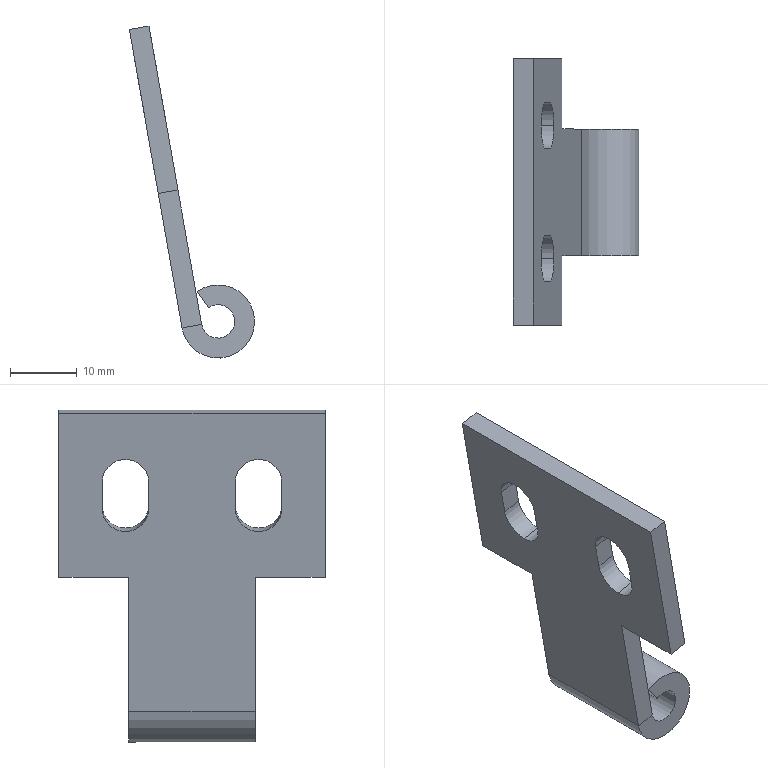Component | SolidWorks | KSHE-016.4-1_Hinge1-1 | 1 solid | 24 faces | box 18.82 x 40 x 49.87 mm | volume 4944 mm3 | plane 16 | cylinder 8 | commonest cylinder face diameters 7 x6 11 x1 5 x1
STEP:
#1=CARTESIAN_POINT('',(-12.205,5.878,2.959));
#2=VERTEX_POINT('',#1);
#3=CARTESIAN_POINT('',(-12.229,5.741,3.094));
#4=VERTEX_POINT('',#3);
#5=CARTESIAN_POINT('',(-12.229,5.878,3.094));
#6=DIRECTION('',(-0.9848,-0.,-0.1736));
#7=DIRECTION('',(0.1736,0.,-0.9848));
#8=AXIS2_PLACEMENT_3D('',#5,#6,#7);
#9=CIRCLE('',#8,0.1378);
#10=EDGE_CURVE('',#2,#4,#9,.T.);
#11=ORIENTED_EDGE('',*,*,#10,.F.);
#12=CARTESIAN_POINT('',(-12.321,5.878,2.938));
#13=VERTEX_POINT('',#12);
#14=CARTESIAN_POINT('',(-11.934,5.878,3.006));
#15=DIRECTION('',(-0.9848,-0.,-0.1736));
#16=VECTOR('',#15,39.37);
#17=LINE('',#14,#16);
#18=EDGE_CURVE('',#2,#13,#17,.T.);
#19=ORIENTED_EDGE('',*,*,#18,.T.);
#20=CARTESIAN_POINT('',(-12.345,5.741,3.074));
#21=VERTEX_POINT('',#20);
#22=CARTESIAN_POINT('',(-12.345,5.878,3.074));
#23=DIRECTION('',(-0.9848,-0.,-0.1736));
#24=DIRECTION('',(0.1736,0.,-0.9848));
#25=AXIS2_PLACEMENT_3D('',#22,#23,#24);
#26=CIRCLE('',#25,0.1378);
#27=EDGE_CURVE('',#13,#21,#26,.T.);
#28=ORIENTED_EDGE('',*,*,#27,.T.);
#29=CARTESIAN_POINT('',(-11.958,5.741,3.142));
#30=DIRECTION('',(-0.9848,-0.,-0.1736));
#31=VECTOR('',#30,39.37);
#32=LINE('',#29,#31);
#33=EDGE_CURVE('',#4,#21,#32,.T.);
#34=ORIENTED_EDGE('',*,*,#33,.F.);
#35=EDGE_LOOP('',(#11,#19,#28,#34));
#36=FACE_OUTER_BOUND('',#35,.T.);
#37=CARTESIAN_POINT('',(-11.958,5.878,3.142));
#38=DIRECTION('',(-0.9848,-0.,-0.1736));
#39=DIRECTION('',(0.1736,0.,-0.9848));
#40=AXIS2_PLACEMENT_3D('',#37,#38,#39);
#41=CYLINDRICAL_SURFACE('',#40,0.1378);
#42=ADVANCED_FACE('',(#36),#41,.F.);
#43=CARTESIAN_POINT('',(-12.205,5.091,2.959));
#44=VERTEX_POINT('',#43);
#45=CARTESIAN_POINT('',(-12.229,4.953,3.094));
#46=VERTEX_POINT('',#45);
#47=CARTESIAN_POINT('',(-12.229,5.091,3.094));
#48=DIRECTION('',(-0.9848,-0.,-0.1736));
#49=DIRECTION('',(0.1736,0.,-0.9848));
#50=AXIS2_PLACEMENT_3D('',#47,#48,#49);
#51=CIRCLE('',#50,0.1378);
#52=EDGE_CURVE('',#44,#46,#51,.T.);
#53=ORIENTED_EDGE('',*,*,#52,.F.);
#54=CARTESIAN_POINT('',(-12.321,5.091,2.938));
#55=VERTEX_POINT('',#54);
#56=CARTESIAN_POINT('',(-11.934,5.091,3.006));
#57=DIRECTION('',(-0.9848,-0.,-0.1736));
#58=VECTOR('',#57,39.37);
#59=LINE('',#56,#58);
#60=EDGE_CURVE('',#44,#55,#59,.T.);
#61=ORIENTED_EDGE('',*,*,#60,.T.);
#62=CARTESIAN_POINT('',(-12.345,4.953,3.074));
#63=VERTEX_POINT('',#62);
#64=CARTESIAN_POINT('',(-12.345,5.091,3.074));
#65=DIRECTION('',(-0.9848,-0.,-0.1736));
#66=DIRECTION('',(0.1736,0.,-0.9848));
#67=AXIS2_PLACEMENT_3D('',#64,#65,#66);
#68=CIRCLE('',#67,0.1378);
#69=EDGE_CURVE('',#55,#63,#68,.T.);
#70=ORIENTED_EDGE('',*,*,#69,.T.);
#71=CARTESIAN_POINT('',(-11.958,4.953,3.142));
#72=DIRECTION('',(-0.9848,-0.,-0.1736));
#73=VECTOR('',#72,39.37);
#74=LINE('',#71,#73);
#75=EDGE_CURVE('',#46,#63,#74,.T.);
#76=ORIENTED_EDGE('',*,*,#75,.F.);
#77=EDGE_LOOP('',(#53,#61,#70,#76));
#78=FACE_OUTER_BOUND('',#77,.T.);
#79=CARTESIAN_POINT('',(-11.958,5.091,3.142));
#80=DIRECTION('',(-0.9848,-0.,-0.1736));
#81=DIRECTION('',(0.1736,0.,-0.9848));
#82=AXIS2_PLACEMENT_3D('',#79,#80,#81);
#83=CYLINDRICAL_SURFACE('',#82,0.1378);
#84=ADVANCED_FACE('',(#78),#83,.F.);
#85=CARTESIAN_POINT('',(-12.274,6.272,2.667));
#86=VERTEX_POINT('',#85);
#87=CARTESIAN_POINT('',(-12.157,6.272,2.687));
#88=VERTEX_POINT('',#87);
#89=CARTESIAN_POINT('',(-12.157,6.272,2.687));
#90=DIRECTION('',(0.9848,0.,0.1736));
#91=VECTOR('',#90,39.37);
#92=LINE('',#89,#91);
#93=EDGE_CURVE('',#86,#88,#92,.T.);
#94=ORIENTED_EDGE('',*,*,#93,.F.);
#95=CARTESIAN_POINT('',(-12.445,6.272,3.636));
#96=VERTEX_POINT('',#95);
#97=CARTESIAN_POINT('',(-12.445,6.272,3.636));
#98=DIRECTION('',(0.1736,-0.,-0.9848));
#99=VECTOR('',#98,39.37);
#100=LINE('',#97,#99);
#101=EDGE_CURVE('',#96,#86,#100,.T.);
#102=ORIENTED_EDGE('',*,*,#101,.F.);
#103=CARTESIAN_POINT('',(-12.328,6.272,3.656));
#104=VERTEX_POINT('',#103);
#105=CARTESIAN_POINT('',(-12.328,6.272,3.656));
#106=DIRECTION('',(-0.9848,-0.,-0.1736));
#107=VECTOR('',#106,39.37);
#108=LINE('',#105,#107);
#109=EDGE_CURVE('',#104,#96,#108,.T.);
#110=ORIENTED_EDGE('',*,*,#109,.F.);
#111=CARTESIAN_POINT('',(-12.328,6.272,3.656));
#112=DIRECTION('',(0.1736,-0.,-0.9848));
#113=VECTOR('',#112,39.37);
#114=LINE('',#111,#113);
#115=EDGE_CURVE('',#104,#88,#114,.T.);
#116=ORIENTED_EDGE('',*,*,#115,.T.);
#117=EDGE_LOOP('',(#94,#102,#110,#116));
#118=FACE_OUTER_BOUND('',#117,.T.);
#119=CARTESIAN_POINT('',(-12.328,6.272,3.656));
#120=DIRECTION('',(-0.,1.,-0.));
#121=DIRECTION('',(0.9848,0.,0.1736));
#122=AXIS2_PLACEMENT_3D('',#119,#120,#121);
#123=PLANE('',#122);
#124=ADVANCED_FACE('',(#118),#123,.T.);
#125=CARTESIAN_POINT('',(-12.445,4.697,3.636));
#126=VERTEX_POINT('',#125);
#127=CARTESIAN_POINT('',(-12.445,4.697,3.636));
#128=DIRECTION('',(-0.,1.,-0.));
#129=VECTOR('',#128,39.37);
#130=LINE('',#127,#129);
#131=EDGE_CURVE('',#126,#96,#130,.T.);
#132=ORIENTED_EDGE('',*,*,#131,.F.);
#133=CARTESIAN_POINT('',(-12.328,4.697,3.656));
#134=VERTEX_POINT('',#133);
#135=CARTESIAN_POINT('',(-12.328,4.697,3.656));
#136=DIRECTION('',(-0.9848,-0.,-0.1736));
#137=VECTOR('',#136,39.37);
#138=LINE('',#135,#137);
#139=EDGE_CURVE('',#134,#126,#138,.T.);
#140=ORIENTED_EDGE('',*,*,#139,.F.);
#141=CARTESIAN_POINT('',(-12.328,4.697,3.656));
#142=DIRECTION('',(-0.,1.,-0.));
#143=VECTOR('',#142,39.37);
#144=LINE('',#141,#143);
#145=EDGE_CURVE('',#134,#104,#144,.T.);
#146=ORIENTED_EDGE('',*,*,#145,.T.);
#147=ORIENTED_EDGE('',*,*,#109,.T.);
#148=EDGE_LOOP('',(#132,#140,#146,#147));
#149=FACE_OUTER_BOUND('',#148,.T.);
#150=CARTESIAN_POINT('',(-12.328,4.697,3.656));
#151=DIRECTION('',(-0.1736,0.,0.9848));
#152=DIRECTION('',(-0.,1.,-0.));
#153=AXIS2_PLACEMENT_3D('',#150,#151,#152);
#154=PLANE('',#153);
#155=ADVANCED_FACE('',(#149),#154,.T.);
#156=CARTESIAN_POINT('',(-12.157,4.697,2.687));
#157=VERTEX_POINT('',#156);
#158=CARTESIAN_POINT('',(-12.274,4.697,2.667));
#159=VERTEX_POINT('',#158);
#160=CARTESIAN_POINT('',(-12.157,4.697,2.687));
#161=DIRECTION('',(-0.9848,-0.,-0.1736));
#162=VECTOR('',#161,39.37);
#163=LINE('',#160,#162);
#164=EDGE_CURVE('',#157,#159,#163,.T.);
#165=ORIENTED_EDGE('',*,*,#164,.F.);
#166=CARTESIAN_POINT('',(-12.328,4.697,3.656));
#167=DIRECTION('',(-0.1736,0.,0.9848));
#168=VECTOR('',#167,39.37);
#169=LINE('',#166,#168);
#170=EDGE_CURVE('',#157,#134,#169,.T.);
#171=ORIENTED_EDGE('',*,*,#170,.T.);
#172=ORIENTED_EDGE('',*,*,#139,.T.);
#173=CARTESIAN_POINT('',(-12.445,4.697,3.636));
#174=DIRECTION('',(-0.1736,0.,0.9848));
#175=VECTOR('',#174,39.37);
#176=LINE('',#173,#175);
#177=EDGE_CURVE('',#159,#126,#176,.T.);
#178=ORIENTED_EDGE('',*,*,#177,.F.);
#179=EDGE_LOOP('',(#165,#171,#172,#178));
#180=FACE_OUTER_BOUND('',#179,.T.);
#181=CARTESIAN_POINT('',(-12.328,4.697,3.656));
#182=DIRECTION('',(0.,-1.,0.));
#183=DIRECTION('',(-0.9848,-0.,-0.1736));
#184=AXIS2_PLACEMENT_3D('',#181,#182,#183);
#185=PLANE('',#184);
#186=ADVANCED_FACE('',(#180),#185,.T.);
#187=CARTESIAN_POINT('',(-12.256,5.741,3.249));
#188=VERTEX_POINT('',#187);
#189=CARTESIAN_POINT('',(-12.154,5.741,2.668));
#190=DIRECTION('',(-0.1736,0.,0.9848));
#191=VECTOR('',#190,39.37);
#192=LINE('',#189,#191);
#193=EDGE_CURVE('',#4,#188,#192,.T.);
#194=ORIENTED_EDGE('',*,*,#193,.T.);
#195=CARTESIAN_POINT('',(-12.256,6.016,3.249));
#196=VERTEX_POINT('',#195);
#197=CARTESIAN_POINT('',(-12.256,5.878,3.249));
#198=DIRECTION('',(-0.9848,-0.,-0.1736));
#199=DIRECTION('',(0.1736,0.,-0.9848));
#200=AXIS2_PLACEMENT_3D('',#197,#198,#199);
#201=CIRCLE('',#200,0.1378);
#202=EDGE_CURVE('',#188,#196,#201,.T.);
#203=ORIENTED_EDGE('',*,*,#202,.T.);
#204=CARTESIAN_POINT('',(-12.229,6.016,3.094));
#205=VERTEX_POINT('',#204);
#206=CARTESIAN_POINT('',(-12.154,6.016,2.668));
#207=DIRECTION('',(0.1736,-0.,-0.9848));
#208=VECTOR('',#207,39.37);
#209=LINE('',#206,#208);
#210=EDGE_CURVE('',#196,#205,#209,.T.);
#211=ORIENTED_EDGE('',*,*,#210,.T.);
#212=CARTESIAN_POINT('',(-12.229,5.878,3.094));
#213=DIRECTION('',(-0.9848,-0.,-0.1736));
#214=DIRECTION('',(0.1736,0.,-0.9848));
#215=AXIS2_PLACEMENT_3D('',#212,#213,#214);
#216=CIRCLE('',#215,0.1378);
#217=EDGE_CURVE('',#205,#2,#216,.T.);
#218=ORIENTED_EDGE('',*,*,#217,.T.);
#219=ORIENTED_EDGE('',*,*,#10,.T.);
#220=EDGE_LOOP('',(#194,#203,#211,#218,#219));
#221=FACE_BOUND('',#220,.T.);
#222=CARTESIAN_POINT('',(-12.256,4.953,3.249));
#223=VERTEX_POINT('',#222);
#224=CARTESIAN_POINT('',(-12.154,4.953,2.668));
#225=DIRECTION('',(-0.1736,0.,0.9848));
#226=VECTOR('',#225,39.37);
#227=LINE('',#224,#226);
#228=EDGE_CURVE('',#46,#223,#227,.T.);
#229=ORIENTED_EDGE('',*,*,#228,.T.);
#230=CARTESIAN_POINT('',(-12.256,5.229,3.249));
#231=VERTEX_POINT('',#230);
#232=CARTESIAN_POINT('',(-12.256,5.091,3.249));
#233=DIRECTION('',(-0.9848,-0.,-0.1736));
#234=DIRECTION('',(0.1736,0.,-0.9848));
#235=AXIS2_PLACEMENT_3D('',#232,#233,#234);
#236=CIRCLE('',#235,0.1378);
#237=EDGE_CURVE('',#223,#231,#236,.T.);
#238=ORIENTED_EDGE('',*,*,#237,.T.);
#239=CARTESIAN_POINT('',(-12.229,5.229,3.094));
#240=VERTEX_POINT('',#239);
#241=CARTESIAN_POINT('',(-12.154,5.229,2.668));
#242=DIRECTION('',(0.1736,-0.,-0.9848));
#243=VECTOR('',#242,39.37);
#244=LINE('',#241,#243);
#245=EDGE_CURVE('',#231,#240,#244,.T.);
#246=ORIENTED_EDGE('',*,*,#245,.T.);
#247=CARTESIAN_POINT('',(-12.229,5.091,3.094));
#248=DIRECTION('',(-0.9848,-0.,-0.1736));
#249=DIRECTION('',(0.1736,0.,-0.9848));
#250=AXIS2_PLACEMENT_3D('',#247,#248,#249);
#251=CIRCLE('',#250,0.1378);
#252=EDGE_CURVE('',#240,#44,#251,.T.);
#253=ORIENTED_EDGE('',*,*,#252,.T.);
#254=ORIENTED_EDGE('',*,*,#52,.T.);
#255=EDGE_LOOP('',(#229,#238,#246,#253,#254));
#256=FACE_BOUND('',#255,.T.);
#257=CARTESIAN_POINT('',(-12.157,5.111,2.687));
#258=VERTEX_POINT('',#257);
#259=CARTESIAN_POINT('',(-12.017,5.111,1.892));
#260=VERTEX_POINT('',#259);
#261=CARTESIAN_POINT('',(-12.154,5.111,2.668));
#262=DIRECTION('',(0.1736,-0.,-0.9848));
#263=VECTOR('',#262,39.37);
#264=LINE('',#261,#263);
#265=EDGE_CURVE('',#258,#260,#264,.T.);
#266=ORIENTED_EDGE('',*,*,#265,.T.);
#267=CARTESIAN_POINT('',(-12.017,5.859,1.892));
#268=VERTEX_POINT('',#267);
#269=CARTESIAN_POINT('',(-12.017,5.859,1.892));
#270=DIRECTION('',(0.,-1.,0.));
#271=VECTOR('',#270,39.37);
#272=LINE('',#269,#271);
#273=EDGE_CURVE('',#268,#260,#272,.T.);
#274=ORIENTED_EDGE('',*,*,#273,.F.);
#275=CARTESIAN_POINT('',(-12.157,5.859,2.687));
#276=VERTEX_POINT('',#275);
#277=CARTESIAN_POINT('',(-12.154,5.859,2.668));
#278=DIRECTION('',(-0.1736,0.,0.9848));
#279=VECTOR('',#278,39.37);
#280=LINE('',#277,#279);
#281=EDGE_CURVE('',#268,#276,#280,.T.);
#282=ORIENTED_EDGE('',*,*,#281,.T.);
#283=CARTESIAN_POINT('',(-12.157,5.485,2.687));
#284=DIRECTION('',(-0.,1.,-0.));
#285=VECTOR('',#284,39.37);
#286=LINE('',#283,#285);
#287=EDGE_CURVE('',#276,#88,#286,.T.);
#288=ORIENTED_EDGE('',*,*,#287,.T.);
#289=ORIENTED_EDGE('',*,*,#115,.F.);
#290=ORIENTED_EDGE('',*,*,#145,.F.);
#291=ORIENTED_EDGE('',*,*,#170,.F.);
#292=CARTESIAN_POINT('',(-12.157,5.485,2.687));
#293=DIRECTION('',(-0.,1.,-0.));
#294=VECTOR('',#293,39.37);
#295=LINE('',#292,#294);
#296=EDGE_CURVE('',#157,#258,#295,.T.);
#297=ORIENTED_EDGE('',*,*,#296,.T.);
#298=EDGE_LOOP('',(#266,#274,#282,#288,#289,#290,#291,#297));
#299=FACE_OUTER_BOUND('',#298,.T.);
#300=CARTESIAN_POINT('',(-12.154,5.485,2.668));
#301=DIRECTION('',(-0.9848,-0.,-0.1736));
#302=DIRECTION('',(0.1736,-0.,-0.9848));
#303=AXIS2_PLACEMENT_3D('',#300,#301,#302);
#304=PLANE('',#303);
#305=ADVANCED_FACE('',(#221,#256,#299),#304,.F.);
#306=CARTESIAN_POINT('',(-12.373,5.741,3.229));
#307=VERTEX_POINT('',#306);
#308=CARTESIAN_POINT('',(-12.373,6.016,3.229));
#309=VERTEX_POINT('',#308);
#310=CARTESIAN_POINT('',(-12.373,5.878,3.229));
#311=DIRECTION('',(-0.9848,-0.,-0.1736));
#312=DIRECTION('',(0.1736,0.,-0.9848));
#313=AXIS2_PLACEMENT_3D('',#310,#311,#312);
#314=CIRCLE('',#313,0.1378);
#315=EDGE_CURVE('',#307,#309,#314,.T.);
#316=ORIENTED_EDGE('',*,*,#315,.F.);
#317=CARTESIAN_POINT('',(-12.373,5.741,3.229));
#318=DIRECTION('',(-0.1736,0.,0.9848));
#319=VECTOR('',#318,39.37);
#320=LINE('',#317,#319);
#321=EDGE_CURVE('',#21,#307,#320,.T.);
#322=ORIENTED_EDGE('',*,*,#321,.F.);
#323=ORIENTED_EDGE('',*,*,#27,.F.);
#324=CARTESIAN_POINT('',(-12.345,6.016,3.074));
#325=VERTEX_POINT('',#324);
#326=CARTESIAN_POINT('',(-12.345,5.878,3.074));
#327=DIRECTION('',(-0.9848,-0.,-0.1736));
#328=DIRECTION('',(0.1736,0.,-0.9848));
#329=AXIS2_PLACEMENT_3D('',#326,#327,#328);
#330=CIRCLE('',#329,0.1378);
#331=EDGE_CURVE('',#325,#13,#330,.T.);
#332=ORIENTED_EDGE('',*,*,#331,.F.);
#333=CARTESIAN_POINT('',(-12.373,6.016,3.229));
#334=DIRECTION('',(0.1736,-0.,-0.9848));
#335=VECTOR('',#334,39.37);
#336=LINE('',#333,#335);
#337=EDGE_CURVE('',#309,#325,#336,.T.);
#338=ORIENTED_EDGE('',*,*,#337,.F.);
#339=EDGE_LOOP('',(#316,#322,#323,#332,#338));
#340=FACE_BOUND('',#339,.T.);
#341=CARTESIAN_POINT('',(-12.373,4.953,3.229));
#342=VERTEX_POINT('',#341);
#343=CARTESIAN_POINT('',(-12.373,5.229,3.229));
#344=VERTEX_POINT('',#343);
#345=CARTESIAN_POINT('',(-12.373,5.091,3.229));
#346=DIRECTION('',(-0.9848,-0.,-0.1736));
#347=DIRECTION('',(0.1736,0.,-0.9848));
#348=AXIS2_PLACEMENT_3D('',#345,#346,#347);
#349=CIRCLE('',#348,0.1378);
#350=EDGE_CURVE('',#342,#344,#349,.T.);
#351=ORIENTED_EDGE('',*,*,#350,.F.);
#352=CARTESIAN_POINT('',(-12.373,4.953,3.229));
#353=DIRECTION('',(-0.1736,0.,0.9848));
#354=VECTOR('',#353,39.37);
#355=LINE('',#352,#354);
#356=EDGE_CURVE('',#63,#342,#355,.T.);
#357=ORIENTED_EDGE('',*,*,#356,.F.);
#358=ORIENTED_EDGE('',*,*,#69,.F.);
#359=CARTESIAN_POINT('',(-12.345,5.229,3.074));
#360=VERTEX_POINT('',#359);
#361=CARTESIAN_POINT('',(-12.345,5.091,3.074));
#362=DIRECTION('',(-0.9848,-0.,-0.1736));
#363=DIRECTION('',(0.1736,0.,-0.9848));
#364=AXIS2_PLACEMENT_3D('',#361,#362,#363);
#365=CIRCLE('',#364,0.1378);
#366=EDGE_CURVE('',#360,#55,#365,.T.);
#367=ORIENTED_EDGE('',*,*,#366,.F.);
#368=CARTESIAN_POINT('',(-12.373,5.229,3.229));
#369=DIRECTION('',(0.1736,-0.,-0.9848));
#370=VECTOR('',#369,39.37);
#371=LINE('',#368,#370);
#372=EDGE_CURVE('',#344,#360,#371,.T.);
#373=ORIENTED_EDGE('',*,*,#372,.F.);
#374=EDGE_LOOP('',(#351,#357,#358,#367,#373));
#375=FACE_BOUND('',#374,.T.);
#376=CARTESIAN_POINT('',(-12.133,5.859,1.872));
#377=VERTEX_POINT('',#376);
#378=CARTESIAN_POINT('',(-12.133,5.111,1.872));
#379=VERTEX_POINT('',#378);
#380=CARTESIAN_POINT('',(-12.133,5.859,1.872));
#381=DIRECTION('',(0.,-1.,0.));
#382=VECTOR('',#381,39.37);
#383=LINE('',#380,#382);
#384=EDGE_CURVE('',#377,#379,#383,.T.);
#385=ORIENTED_EDGE('',*,*,#384,.T.);
#386=CARTESIAN_POINT('',(-12.274,5.111,2.667));
#387=VERTEX_POINT('',#386);
#388=CARTESIAN_POINT('',(-12.274,5.111,2.667));
#389=DIRECTION('',(0.1736,-0.,-0.9848));
#390=VECTOR('',#389,39.37);
#391=LINE('',#388,#390);
#392=EDGE_CURVE('',#387,#379,#391,.T.);
#393=ORIENTED_EDGE('',*,*,#392,.F.);
#394=CARTESIAN_POINT('',(-12.274,5.485,2.667));
#395=DIRECTION('',(-0.,1.,-0.));
#396=VECTOR('',#395,39.37);
#397=LINE('',#394,#396);
#398=EDGE_CURVE('',#159,#387,#397,.T.);
#399=ORIENTED_EDGE('',*,*,#398,.F.);
#400=ORIENTED_EDGE('',*,*,#177,.T.);
#401=ORIENTED_EDGE('',*,*,#131,.T.);
#402=ORIENTED_EDGE('',*,*,#101,.T.);
#403=CARTESIAN_POINT('',(-12.274,5.859,2.667));
#404=VERTEX_POINT('',#403);
#405=CARTESIAN_POINT('',(-12.274,5.859,2.667));
#406=DIRECTION('',(-0.,1.,-0.));
#407=VECTOR('',#406,39.37);
#408=LINE('',#405,#407);
#409=EDGE_CURVE('',#404,#86,#408,.T.);
#410=ORIENTED_EDGE('',*,*,#409,.F.);
#411=CARTESIAN_POINT('',(-12.27,5.859,2.647));
#412=DIRECTION('',(-0.1736,0.,0.9848));
#413=VECTOR('',#412,39.37);
#414=LINE('',#411,#413);
#415=EDGE_CURVE('',#377,#404,#414,.T.);
#416=ORIENTED_EDGE('',*,*,#415,.F.);
#417=EDGE_LOOP('',(#385,#393,#399,#400,#401,#402,#410,#416));
#418=FACE_OUTER_BOUND('',#417,.T.);
#419=CARTESIAN_POINT('',(-12.27,5.485,2.647));
#420=DIRECTION('',(-0.9848,-0.,-0.1736));
#421=DIRECTION('',(0.1736,-0.,-0.9848));
#422=AXIS2_PLACEMENT_3D('',#419,#420,#421);
#423=PLANE('',#422);
#424=ADVANCED_FACE('',(#340,#375,#418),#423,.T.);
#425=ORIENTED_EDGE('',*,*,#392,.T.);
#426=CARTESIAN_POINT('',(-12.017,5.111,1.892));
#427=DIRECTION('',(-0.9848,-0.,-0.1736));
#428=VECTOR('',#427,39.37);
#429=LINE('',#426,#428);
#430=EDGE_CURVE('',#260,#379,#429,.T.);
#431=ORIENTED_EDGE('',*,*,#430,.F.);
#432=ORIENTED_EDGE('',*,*,#265,.F.);
#433=CARTESIAN_POINT('',(-11.886,5.111,2.735));
#434=DIRECTION('',(-0.9848,-0.,-0.1736));
#435=VECTOR('',#434,39.37);
#436=LINE('',#433,#435);
#437=EDGE_CURVE('',#258,#387,#436,.T.);
#438=ORIENTED_EDGE('',*,*,#437,.T.);
#439=EDGE_LOOP('',(#425,#431,#432,#438));
#440=FACE_OUTER_BOUND('',#439,.T.);
#441=CARTESIAN_POINT('',(-11.886,5.111,2.735));
#442=DIRECTION('',(-0.,1.,-0.));
#443=DIRECTION('',(0.9848,0.,0.1736));
#444=AXIS2_PLACEMENT_3D('',#441,#442,#443);
#445=PLANE('',#444);
#446=ADVANCED_FACE('',(#440),#445,.F.);
#447=ORIENTED_EDGE('',*,*,#164,.T.);
#448=ORIENTED_EDGE('',*,*,#398,.T.);
#449=ORIENTED_EDGE('',*,*,#437,.F.);
#450=ORIENTED_EDGE('',*,*,#296,.F.);
#451=EDGE_LOOP('',(#447,#448,#449,#450));
#452=FACE_OUTER_BOUND('',#451,.T.);
#453=CARTESIAN_POINT('',(-11.886,4.284,2.735));
#454=DIRECTION('',(-0.1736,0.,0.9848));
#455=DIRECTION('',(-0.9848,-0.,-0.1736));
#456=AXIS2_PLACEMENT_3D('',#453,#454,#455);
#457=PLANE('',#456);
#458=ADVANCED_FACE('',(#452),#457,.F.);
#459=ORIENTED_EDGE('',*,*,#93,.T.);
#460=ORIENTED_EDGE('',*,*,#287,.F.);
#461=CARTESIAN_POINT('',(-11.886,5.859,2.735));
#462=DIRECTION('',(-0.9848,-0.,-0.1736));
#463=VECTOR('',#462,39.37);
#464=LINE('',#461,#463);
#465=EDGE_CURVE('',#276,#404,#464,.T.);
#466=ORIENTED_EDGE('',*,*,#465,.T.);
#467=ORIENTED_EDGE('',*,*,#409,.T.);
#468=EDGE_LOOP('',(#459,#460,#466,#467));
#469=FACE_OUTER_BOUND('',#468,.T.);
#470=CARTESIAN_POINT('',(-11.886,5.859,2.735));
#471=DIRECTION('',(-0.1736,0.,0.9848));
#472=DIRECTION('',(-0.9848,-0.,-0.1736));
#473=AXIS2_PLACEMENT_3D('',#470,#471,#472);
#474=PLANE('',#473);
#475=ADVANCED_FACE('',(#469),#474,.F.);
#476=ORIENTED_EDGE('',*,*,#281,.F.);
#477=CARTESIAN_POINT('',(-12.017,5.859,1.892));
#478=DIRECTION('',(-0.9848,-0.,-0.1736));
#479=VECTOR('',#478,39.37);
#480=LINE('',#477,#479);
#481=EDGE_CURVE('',#268,#377,#480,.T.);
#482=ORIENTED_EDGE('',*,*,#481,.T.);
#483=ORIENTED_EDGE('',*,*,#415,.T.);
#484=ORIENTED_EDGE('',*,*,#465,.F.);
#485=EDGE_LOOP('',(#476,#482,#483,#484));
#486=FACE_OUTER_BOUND('',#485,.T.);
#487=CARTESIAN_POINT('',(-11.886,5.859,2.735));
#488=DIRECTION('',(0.,-1.,0.));
#489=DIRECTION('',(-0.9848,-0.,-0.1736));
#490=AXIS2_PLACEMENT_3D('',#487,#488,#489);
#491=PLANE('',#490);
#492=ADVANCED_FACE('',(#486),#491,.F.);
#493=CARTESIAN_POINT('',(-11.977,5.859,1.99));
#494=VERTEX_POINT('',#493);
#495=CARTESIAN_POINT('',(-12.044,5.859,2.087));
#496=VERTEX_POINT('',#495);
#497=CARTESIAN_POINT('',(-11.977,5.859,1.99));
#498=DIRECTION('',(-0.5736,-0.,0.8192));
#499=VECTOR('',#498,39.37);
#500=LINE('',#497,#499);
#501=EDGE_CURVE('',#494,#496,#500,.T.);
#502=ORIENTED_EDGE('',*,*,#501,.F.);
#503=CARTESIAN_POINT('',(-11.977,5.111,1.99));
#504=VERTEX_POINT('',#503);
#505=CARTESIAN_POINT('',(-11.977,5.859,1.99));
#506=DIRECTION('',(-0.,1.,-0.));
#507=VECTOR('',#506,39.37);
#508=LINE('',#505,#507);
#509=EDGE_CURVE('',#504,#494,#508,.T.);
#510=ORIENTED_EDGE('',*,*,#509,.F.);
#511=CARTESIAN_POINT('',(-12.044,5.111,2.087));
#512=VERTEX_POINT('',#511);
#513=CARTESIAN_POINT('',(-11.977,5.111,1.99));
#514=DIRECTION('',(-0.5736,-0.,0.8192));
#515=VECTOR('',#514,39.37);
#516=LINE('',#513,#515);
#517=EDGE_CURVE('',#504,#512,#516,.T.);
#518=ORIENTED_EDGE('',*,*,#517,.T.);
#519=CARTESIAN_POINT('',(-12.044,5.859,2.087));
#520=DIRECTION('',(-0.,1.,-0.));
#521=VECTOR('',#520,39.37);
#522=LINE('',#519,#521);
#523=EDGE_CURVE('',#512,#496,#522,.T.);
#524=ORIENTED_EDGE('',*,*,#523,.T.);
#525=EDGE_LOOP('',(#502,#510,#518,#524));
#526=FACE_OUTER_BOUND('',#525,.T.);
#527=CARTESIAN_POINT('',(-11.977,5.485,1.99));
#528=DIRECTION('',(0.8192,0.,0.5736));
#529=DIRECTION('',(-0.,1.,-0.));
#530=AXIS2_PLACEMENT_3D('',#527,#528,#529);
#531=PLANE('',#530);
#532=ADVANCED_FACE('',(#526),#531,.F.);
#533=ORIENTED_EDGE('',*,*,#517,.F.);
#534=CARTESIAN_POINT('',(-11.92,5.111,1.909));
#535=DIRECTION('',(0.,-1.,0.));
#536=DIRECTION('',(0.9848,0.,0.1736));
#537=AXIS2_PLACEMENT_3D('',#534,#535,#536);
#538=CIRCLE('',#537,0.09843);
#539=EDGE_CURVE('',#260,#504,#538,.T.);
#540=ORIENTED_EDGE('',*,*,#539,.F.);
#541=ORIENTED_EDGE('',*,*,#430,.T.);
#542=CARTESIAN_POINT('',(-11.92,5.111,1.909));
#543=DIRECTION('',(0.,-1.,0.));
#544=DIRECTION('',(0.9848,0.,0.1736));
#545=AXIS2_PLACEMENT_3D('',#542,#543,#544);
#546=CIRCLE('',#545,0.2165);
#547=EDGE_CURVE('',#379,#512,#546,.T.);
#548=ORIENTED_EDGE('',*,*,#547,.T.);
#549=EDGE_LOOP('',(#533,#540,#541,#548));
#550=FACE_OUTER_BOUND('',#549,.T.);
#551=CARTESIAN_POINT('',(-11.92,5.111,1.909));
#552=DIRECTION('',(0.,-1.,0.));
#553=DIRECTION('',(-0.9848,-0.,-0.1736));
#554=AXIS2_PLACEMENT_3D('',#551,#552,#553);
#555=PLANE('',#554);
#556=ADVANCED_FACE('',(#550),#555,.T.);
#557=CARTESIAN_POINT('',(-11.92,5.859,1.909));
#558=DIRECTION('',(-0.,1.,-0.));
#559=DIRECTION('',(0.9848,0.,0.1736));
#560=AXIS2_PLACEMENT_3D('',#557,#558,#559);
#561=CIRCLE('',#560,0.09843);
#562=EDGE_CURVE('',#494,#268,#561,.T.);
#563=ORIENTED_EDGE('',*,*,#562,.F.);
#564=ORIENTED_EDGE('',*,*,#501,.T.);
#565=CARTESIAN_POINT('',(-11.92,5.859,1.909));
#566=DIRECTION('',(-0.,1.,-0.));
#567=DIRECTION('',(0.9848,0.,0.1736));
#568=AXIS2_PLACEMENT_3D('',#565,#566,#567);
#569=CIRCLE('',#568,0.2165);
#570=EDGE_CURVE('',#496,#377,#569,.T.);
#571=ORIENTED_EDGE('',*,*,#570,.T.);
#572=ORIENTED_EDGE('',*,*,#481,.F.);
#573=EDGE_LOOP('',(#563,#564,#571,#572));
#574=FACE_OUTER_BOUND('',#573,.T.);
#575=CARTESIAN_POINT('',(-11.92,5.859,1.909));
#576=DIRECTION('',(0.,-1.,0.));
#577=DIRECTION('',(-0.9848,-0.,-0.1736));
#578=AXIS2_PLACEMENT_3D('',#575,#576,#577);
#579=PLANE('',#578);
#580=ADVANCED_FACE('',(#574),#579,.F.);
#581=ORIENTED_EDGE('',*,*,#384,.F.);
#582=ORIENTED_EDGE('',*,*,#570,.F.);
#583=ORIENTED_EDGE('',*,*,#523,.F.);
#584=ORIENTED_EDGE('',*,*,#547,.F.);
#585=EDGE_LOOP('',(#581,#582,#583,#584));
#586=FACE_OUTER_BOUND('',#585,.T.);
#587=CARTESIAN_POINT('',(-11.92,5.859,1.909));
#588=DIRECTION('',(-0.,1.,-0.));
#589=DIRECTION('',(-0.5736,0.,0.8192));
#590=AXIS2_PLACEMENT_3D('',#587,#588,#589);
#591=CYLINDRICAL_SURFACE('',#590,0.2165);
#592=ADVANCED_FACE('',(#586),#591,.T.);
#593=ORIENTED_EDGE('',*,*,#273,.T.);
#594=ORIENTED_EDGE('',*,*,#539,.T.);
#595=ORIENTED_EDGE('',*,*,#509,.T.);
#596=ORIENTED_EDGE('',*,*,#562,.T.);
#597=EDGE_LOOP('',(#593,#594,#595,#596));
#598=FACE_OUTER_BOUND('',#597,.T.);
#599=CARTESIAN_POINT('',(-11.92,5.859,1.909));
#600=DIRECTION('',(-0.,1.,-0.));
#601=DIRECTION('',(-0.5736,0.,0.8192));
#602=AXIS2_PLACEMENT_3D('',#599,#600,#601);
#603=CYLINDRICAL_SURFACE('',#602,0.09843);
#604=ADVANCED_FACE('',(#598),#603,.F.);
#605=CARTESIAN_POINT('',(-11.985,4.953,3.297));
#606=DIRECTION('',(-0.9848,-0.,-0.1736));
#607=VECTOR('',#606,39.37);
#608=LINE('',#605,#607);
#609=EDGE_CURVE('',#223,#342,#608,.T.);
#610=ORIENTED_EDGE('',*,*,#609,.T.);
#611=ORIENTED_EDGE('',*,*,#350,.T.);
#612=CARTESIAN_POINT('',(-11.985,5.229,3.297));
#613=DIRECTION('',(-0.9848,-0.,-0.1736));
#614=VECTOR('',#613,39.37);
#615=LINE('',#612,#614);
#616=EDGE_CURVE('',#231,#344,#615,.T.);
#617=ORIENTED_EDGE('',*,*,#616,.F.);
#618=ORIENTED_EDGE('',*,*,#237,.F.);
#619=EDGE_LOOP('',(#610,#611,#617,#618));
#620=FACE_OUTER_BOUND('',#619,.T.);
#621=CARTESIAN_POINT('',(-11.985,5.091,3.297));
#622=DIRECTION('',(-0.9848,-0.,-0.1736));
#623=DIRECTION('',(0.1736,0.,-0.9848));
#624=AXIS2_PLACEMENT_3D('',#621,#622,#623);
#625=CYLINDRICAL_SURFACE('',#624,0.1378);
#626=ADVANCED_FACE('',(#620),#625,.F.);
#627=ORIENTED_EDGE('',*,*,#75,.T.);
#628=ORIENTED_EDGE('',*,*,#356,.T.);
#629=ORIENTED_EDGE('',*,*,#609,.F.);
#630=ORIENTED_EDGE('',*,*,#228,.F.);
#631=EDGE_LOOP('',(#627,#628,#629,#630));
#632=FACE_OUTER_BOUND('',#631,.T.);
#633=CARTESIAN_POINT('',(-11.985,4.953,3.297));
#634=DIRECTION('',(0.,-1.,0.));
#635=DIRECTION('',(-0.9848,-0.,-0.1736));
#636=AXIS2_PLACEMENT_3D('',#633,#634,#635);
#637=PLANE('',#636);
#638=ADVANCED_FACE('',(#632),#637,.F.);
#639=ORIENTED_EDGE('',*,*,#60,.F.);
#640=ORIENTED_EDGE('',*,*,#252,.F.);
#641=CARTESIAN_POINT('',(-11.958,5.229,3.142));
#642=DIRECTION('',(-0.9848,-0.,-0.1736));
#643=VECTOR('',#642,39.37);
#644=LINE('',#641,#643);
#645=EDGE_CURVE('',#240,#360,#644,.T.);
#646=ORIENTED_EDGE('',*,*,#645,.T.);
#647=ORIENTED_EDGE('',*,*,#366,.T.);
#648=EDGE_LOOP('',(#639,#640,#646,#647));
#649=FACE_OUTER_BOUND('',#648,.T.);
#650=CARTESIAN_POINT('',(-11.958,5.091,3.142));
#651=DIRECTION('',(-0.9848,-0.,-0.1736));
#652=DIRECTION('',(0.1736,0.,-0.9848));
#653=AXIS2_PLACEMENT_3D('',#650,#651,#652);
#654=CYLINDRICAL_SURFACE('',#653,0.1378);
#655=ADVANCED_FACE('',(#649),#654,.F.);
#656=ORIENTED_EDGE('',*,*,#616,.T.);
#657=ORIENTED_EDGE('',*,*,#372,.T.);
#658=ORIENTED_EDGE('',*,*,#645,.F.);
#659=ORIENTED_EDGE('',*,*,#245,.F.);
#660=EDGE_LOOP('',(#656,#657,#658,#659));
#661=FACE_OUTER_BOUND('',#660,.T.);
#662=CARTESIAN_POINT('',(-11.985,5.229,3.297));
#663=DIRECTION('',(-0.,1.,-0.));
#664=DIRECTION('',(0.1736,-0.,-0.9848));
#665=AXIS2_PLACEMENT_3D('',#662,#663,#664);
#666=PLANE('',#665);
#667=ADVANCED_FACE('',(#661),#666,.F.);
#668=CARTESIAN_POINT('',(-11.985,5.741,3.297));
#669=DIRECTION('',(-0.9848,-0.,-0.1736));
#670=VECTOR('',#669,39.37);
#671=LINE('',#668,#670);
#672=EDGE_CURVE('',#188,#307,#671,.T.);
#673=ORIENTED_EDGE('',*,*,#672,.T.);
#674=ORIENTED_EDGE('',*,*,#315,.T.);
#675=CARTESIAN_POINT('',(-11.985,6.016,3.297));
#676=DIRECTION('',(-0.9848,-0.,-0.1736));
#677=VECTOR('',#676,39.37);
#678=LINE('',#675,#677);
#679=EDGE_CURVE('',#196,#309,#678,.T.);
#680=ORIENTED_EDGE('',*,*,#679,.F.);
#681=ORIENTED_EDGE('',*,*,#202,.F.);
#682=EDGE_LOOP('',(#673,#674,#680,#681));
#683=FACE_OUTER_BOUND('',#682,.T.);
#684=CARTESIAN_POINT('',(-11.985,5.878,3.297));
#685=DIRECTION('',(-0.9848,-0.,-0.1736));
#686=DIRECTION('',(0.1736,0.,-0.9848));
#687=AXIS2_PLACEMENT_3D('',#684,#685,#686);
#688=CYLINDRICAL_SURFACE('',#687,0.1378);
#689=ADVANCED_FACE('',(#683),#688,.F.);
#690=ORIENTED_EDGE('',*,*,#33,.T.);
#691=ORIENTED_EDGE('',*,*,#321,.T.);
#692=ORIENTED_EDGE('',*,*,#672,.F.);
#693=ORIENTED_EDGE('',*,*,#193,.F.);
#694=EDGE_LOOP('',(#690,#691,#692,#693));
#695=FACE_OUTER_BOUND('',#694,.T.);
#696=CARTESIAN_POINT('',(-11.985,5.741,3.297));
#697=DIRECTION('',(0.,-1.,0.));
#698=DIRECTION('',(-0.9848,-0.,-0.1736));
#699=AXIS2_PLACEMENT_3D('',#696,#697,#698);
#700=PLANE('',#699);
#701=ADVANCED_FACE('',(#695),#700,.F.);
#702=ORIENTED_EDGE('',*,*,#18,.F.);
#703=ORIENTED_EDGE('',*,*,#217,.F.);
#704=CARTESIAN_POINT('',(-11.958,6.016,3.142));
#705=DIRECTION('',(-0.9848,-0.,-0.1736));
#706=VECTOR('',#705,39.37);
#707=LINE('',#704,#706);
#708=EDGE_CURVE('',#205,#325,#707,.T.);
#709=ORIENTED_EDGE('',*,*,#708,.T.);
#710=ORIENTED_EDGE('',*,*,#331,.T.);
#711=EDGE_LOOP('',(#702,#703,#709,#710));
#712=FACE_OUTER_BOUND('',#711,.T.);
#713=CARTESIAN_POINT('',(-11.958,5.878,3.142));
#714=DIRECTION('',(-0.9848,-0.,-0.1736));
#715=DIRECTION('',(0.1736,0.,-0.9848));
#716=AXIS2_PLACEMENT_3D('',#713,#714,#715);
#717=CYLINDRICAL_SURFACE('',#716,0.1378);
#718=ADVANCED_FACE('',(#712),#717,.F.);
#719=ORIENTED_EDGE('',*,*,#679,.T.);
#720=ORIENTED_EDGE('',*,*,#337,.T.);
#721=ORIENTED_EDGE('',*,*,#708,.F.);
#722=ORIENTED_EDGE('',*,*,#210,.F.);
#723=EDGE_LOOP('',(#719,#720,#721,#722));
#724=FACE_OUTER_BOUND('',#723,.T.);
#725=CARTESIAN_POINT('',(-11.985,6.016,3.297));
#726=DIRECTION('',(-0.,1.,-0.));
#727=DIRECTION('',(0.9848,0.,0.1736));
#728=AXIS2_PLACEMENT_3D('',#725,#726,#727);
#729=PLANE('',#728);
#730=ADVANCED_FACE('',(#724),#729,.F.);
#731=CLOSED_SHELL('',(#42,#84,#124,#155,#186,#305,#424,#446,#458,#475,#492,#532,#556,#580,#592,#604,#626,#638,#655,#667,#689,#701,#718,#730));
#732=MANIFOLD_SOLID_BREP('',#731);
#733=CARTESIAN_POINT('',(0.,0.,0.));
#734=DIRECTION('',(0.,0.,1.));
#735=DIRECTION('',(1.,0.,0.));
#736=AXIS2_PLACEMENT_3D('',#733,#734,#735);
#737=(LENGTH_UNIT()NAMED_UNIT(*)SI_UNIT($,.METRE.));
#738=LENGTH_MEASURE_WITH_UNIT(LENGTH_MEASURE(0.0254),#737);
#739=DIMENSIONAL_EXPONENTS(1.,0.,0.,0.,0.,0.,0.);
#740=(CONVERSION_BASED_UNIT('',#738)LENGTH_UNIT()NAMED_UNIT(#739));
#741=UNCERTAINTY_MEASURE_WITH_UNIT(LENGTH_MEASURE(0.00001),#740,'','');
#742=(NAMED_UNIT(*)PLANE_ANGLE_UNIT()SI_UNIT($,.RADIAN.));
#743=(NAMED_UNIT(*)SI_UNIT($,.STERADIAN.)SOLID_ANGLE_UNIT());
#744=(GEOMETRIC_REPRESENTATION_CONTEXT(3)GLOBAL_UNCERTAINTY_ASSIGNED_CONTEXT((#741))GLOBAL_UNIT_ASSIGNED_CONTEXT((#740,#742,#743))REPRESENTATION_CONTEXT('',''));
#745=ADVANCED_BREP_SHAPE_REPRESENTATION('',(#732,#736),#744);
#746=COLOUR_RGB('',0.7922,0.8196,0.9333);
#747=FILL_AREA_STYLE_COLOUR('',#746);
#748=FILL_AREA_STYLE('',(#747));
#749=SURFACE_STYLE_FILL_AREA(#748);
#750=SURFACE_SIDE_STYLE('',(#749));
#751=SURFACE_STYLE_USAGE(.BOTH.,#750);
#752=PRESENTATION_STYLE_ASSIGNMENT((#751));
#753=STYLED_ITEM('',(#752),#732);
#754=(LENGTH_UNIT()NAMED_UNIT(*)SI_UNIT($,.METRE.));
#755=LENGTH_MEASURE_WITH_UNIT(LENGTH_MEASURE(0.0254),#754);
#756=DIMENSIONAL_EXPONENTS(1.,0.,0.,0.,0.,0.,0.);
#757=(CONVERSION_BASED_UNIT('',#755)LENGTH_UNIT()NAMED_UNIT(#756));
#758=UNCERTAINTY_MEASURE_WITH_UNIT(LENGTH_MEASURE(0.00001),#757,'','');
#759=(NAMED_UNIT(*)PLANE_ANGLE_UNIT()SI_UNIT($,.RADIAN.));
#760=(NAMED_UNIT(*)SI_UNIT($,.STERADIAN.)SOLID_ANGLE_UNIT());
#761=(GEOMETRIC_REPRESENTATION_CONTEXT(3)GLOBAL_UNCERTAINTY_ASSIGNED_CONTEXT((#758))GLOBAL_UNIT_ASSIGNED_CONTEXT((#757,#759,#760))REPRESENTATION_CONTEXT('',''));
#762=MECHANICAL_DESIGN_GEOMETRIC_PRESENTATION_REPRESENTATION('',(#753),#761);
#763=PRESENTATION_LAYER_ASSIGNMENT('','',(#753));